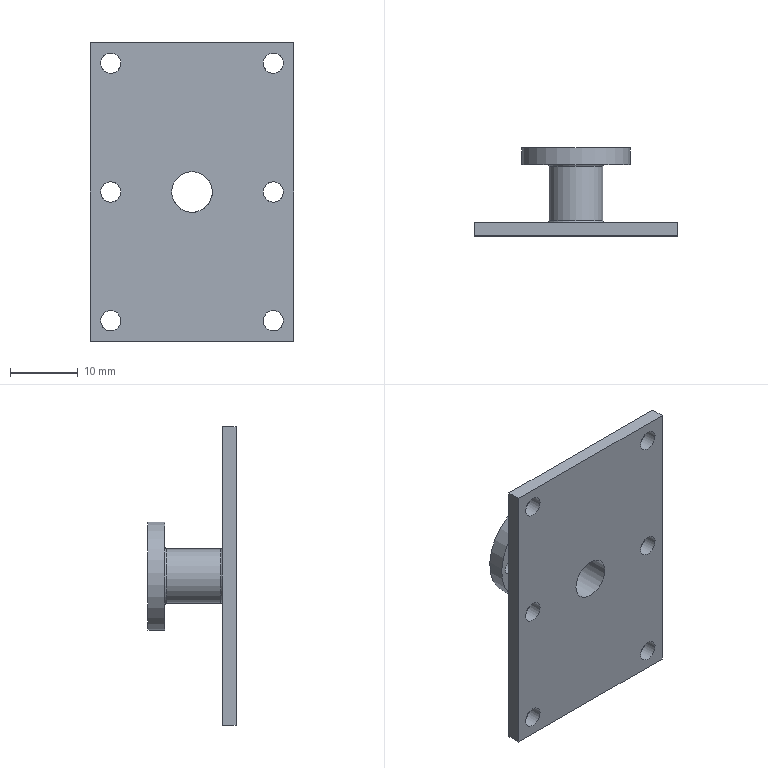Component | NX | AIR_CYLINDER_CONN_PLATE | 1 solid | 23 faces | volume 3069 mm3 | cylinder 13 | plane 8 | torus 2 | commonest cylinder face diameters 3 x6 2.5 x4 8 x1 16 x1 6 x1